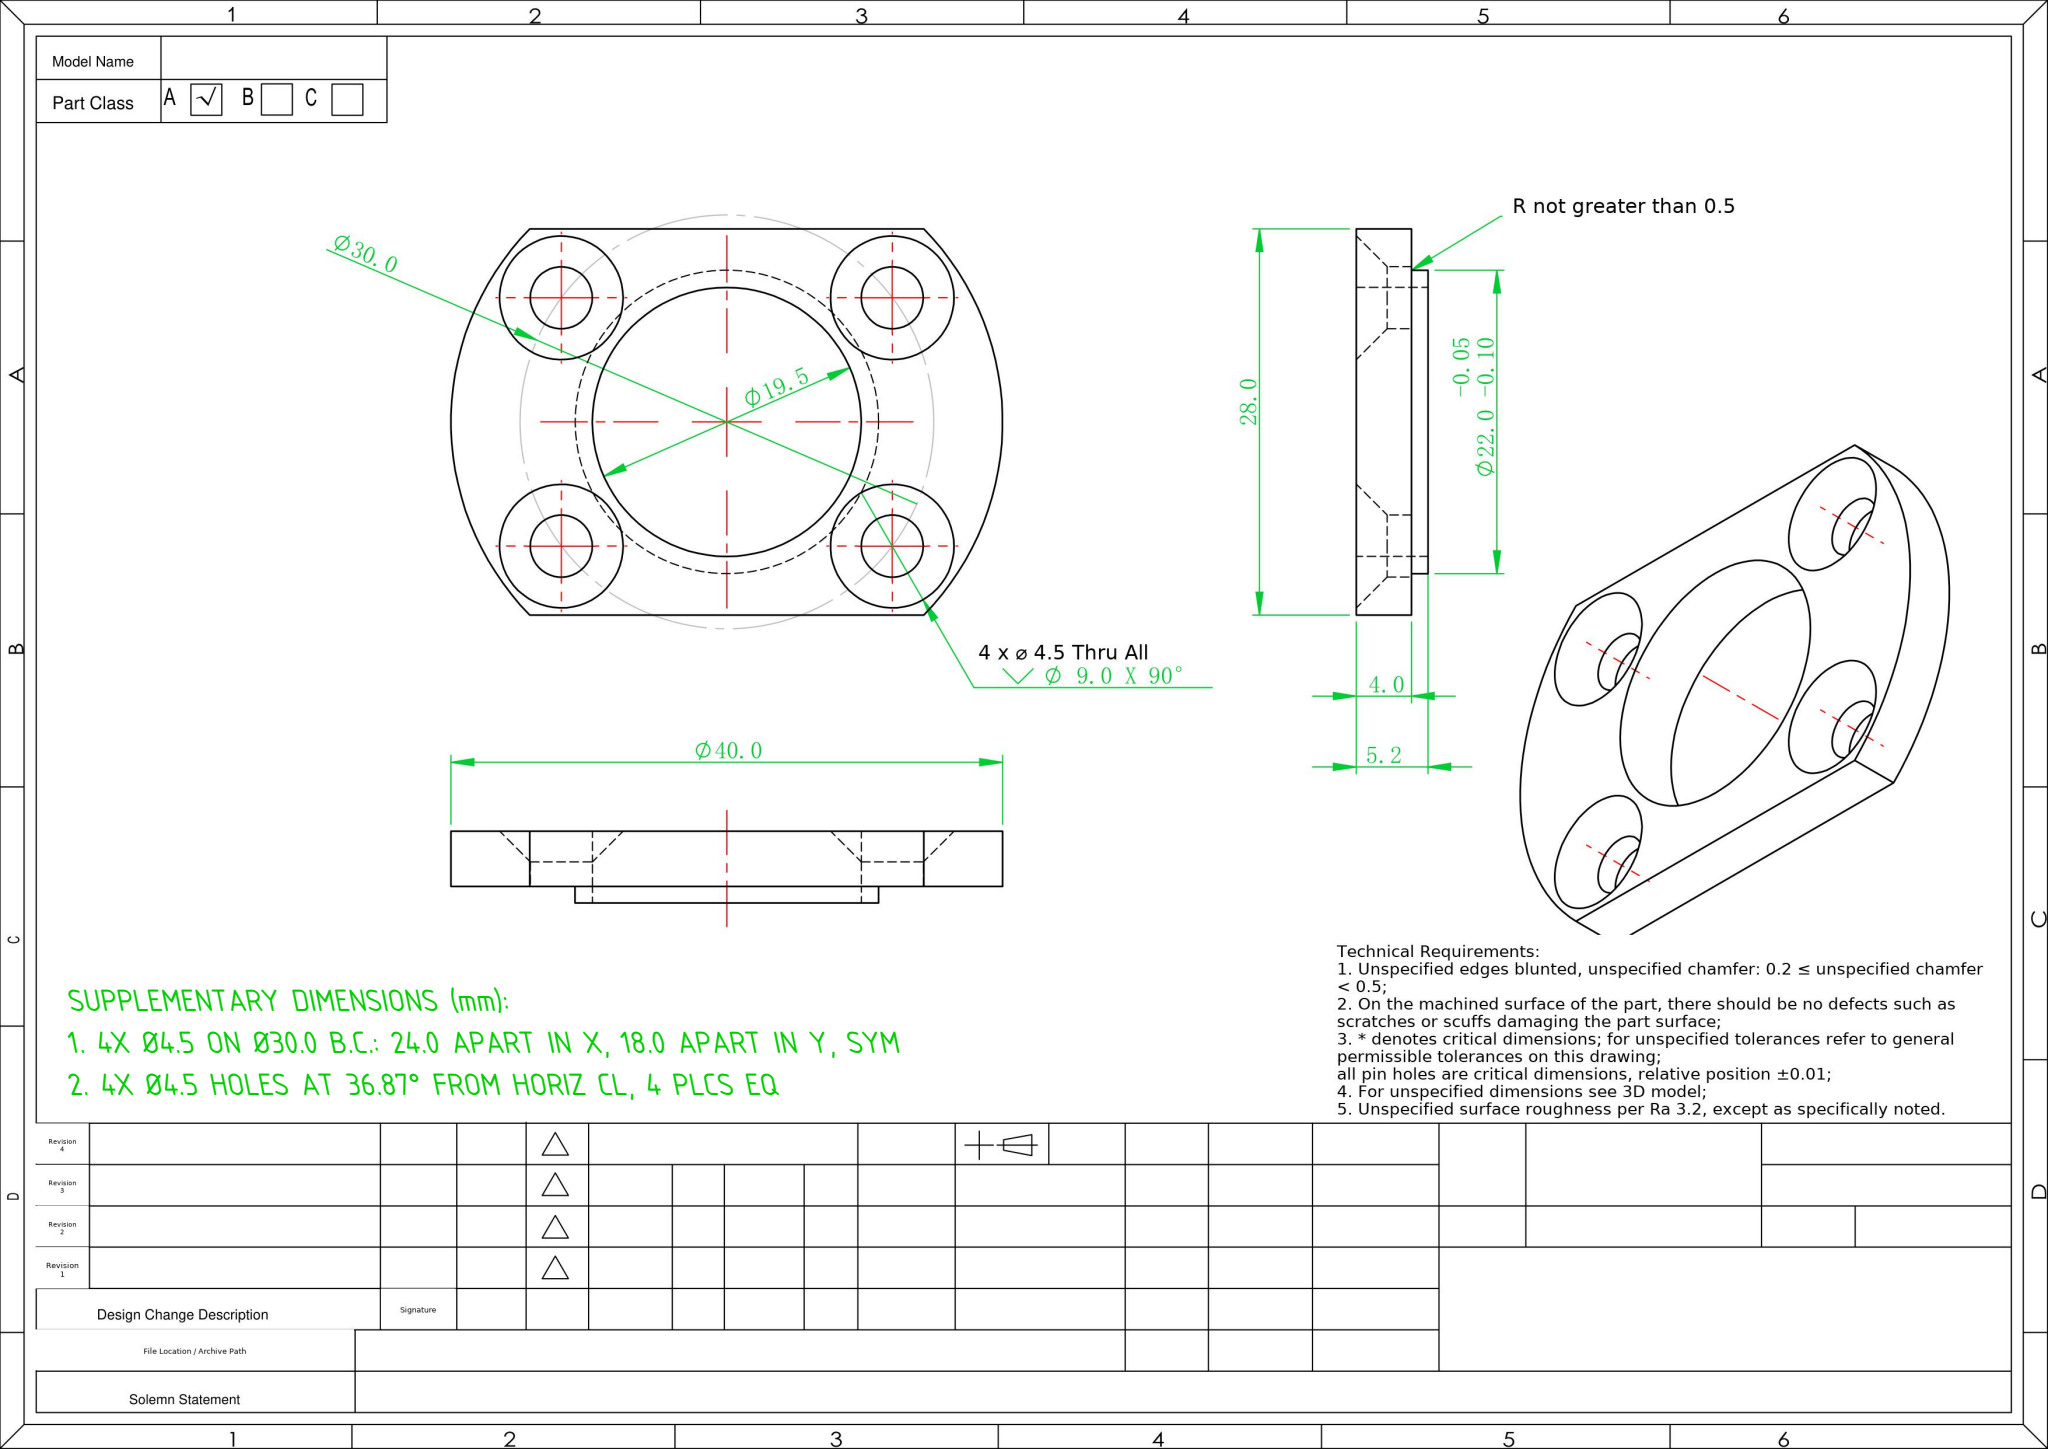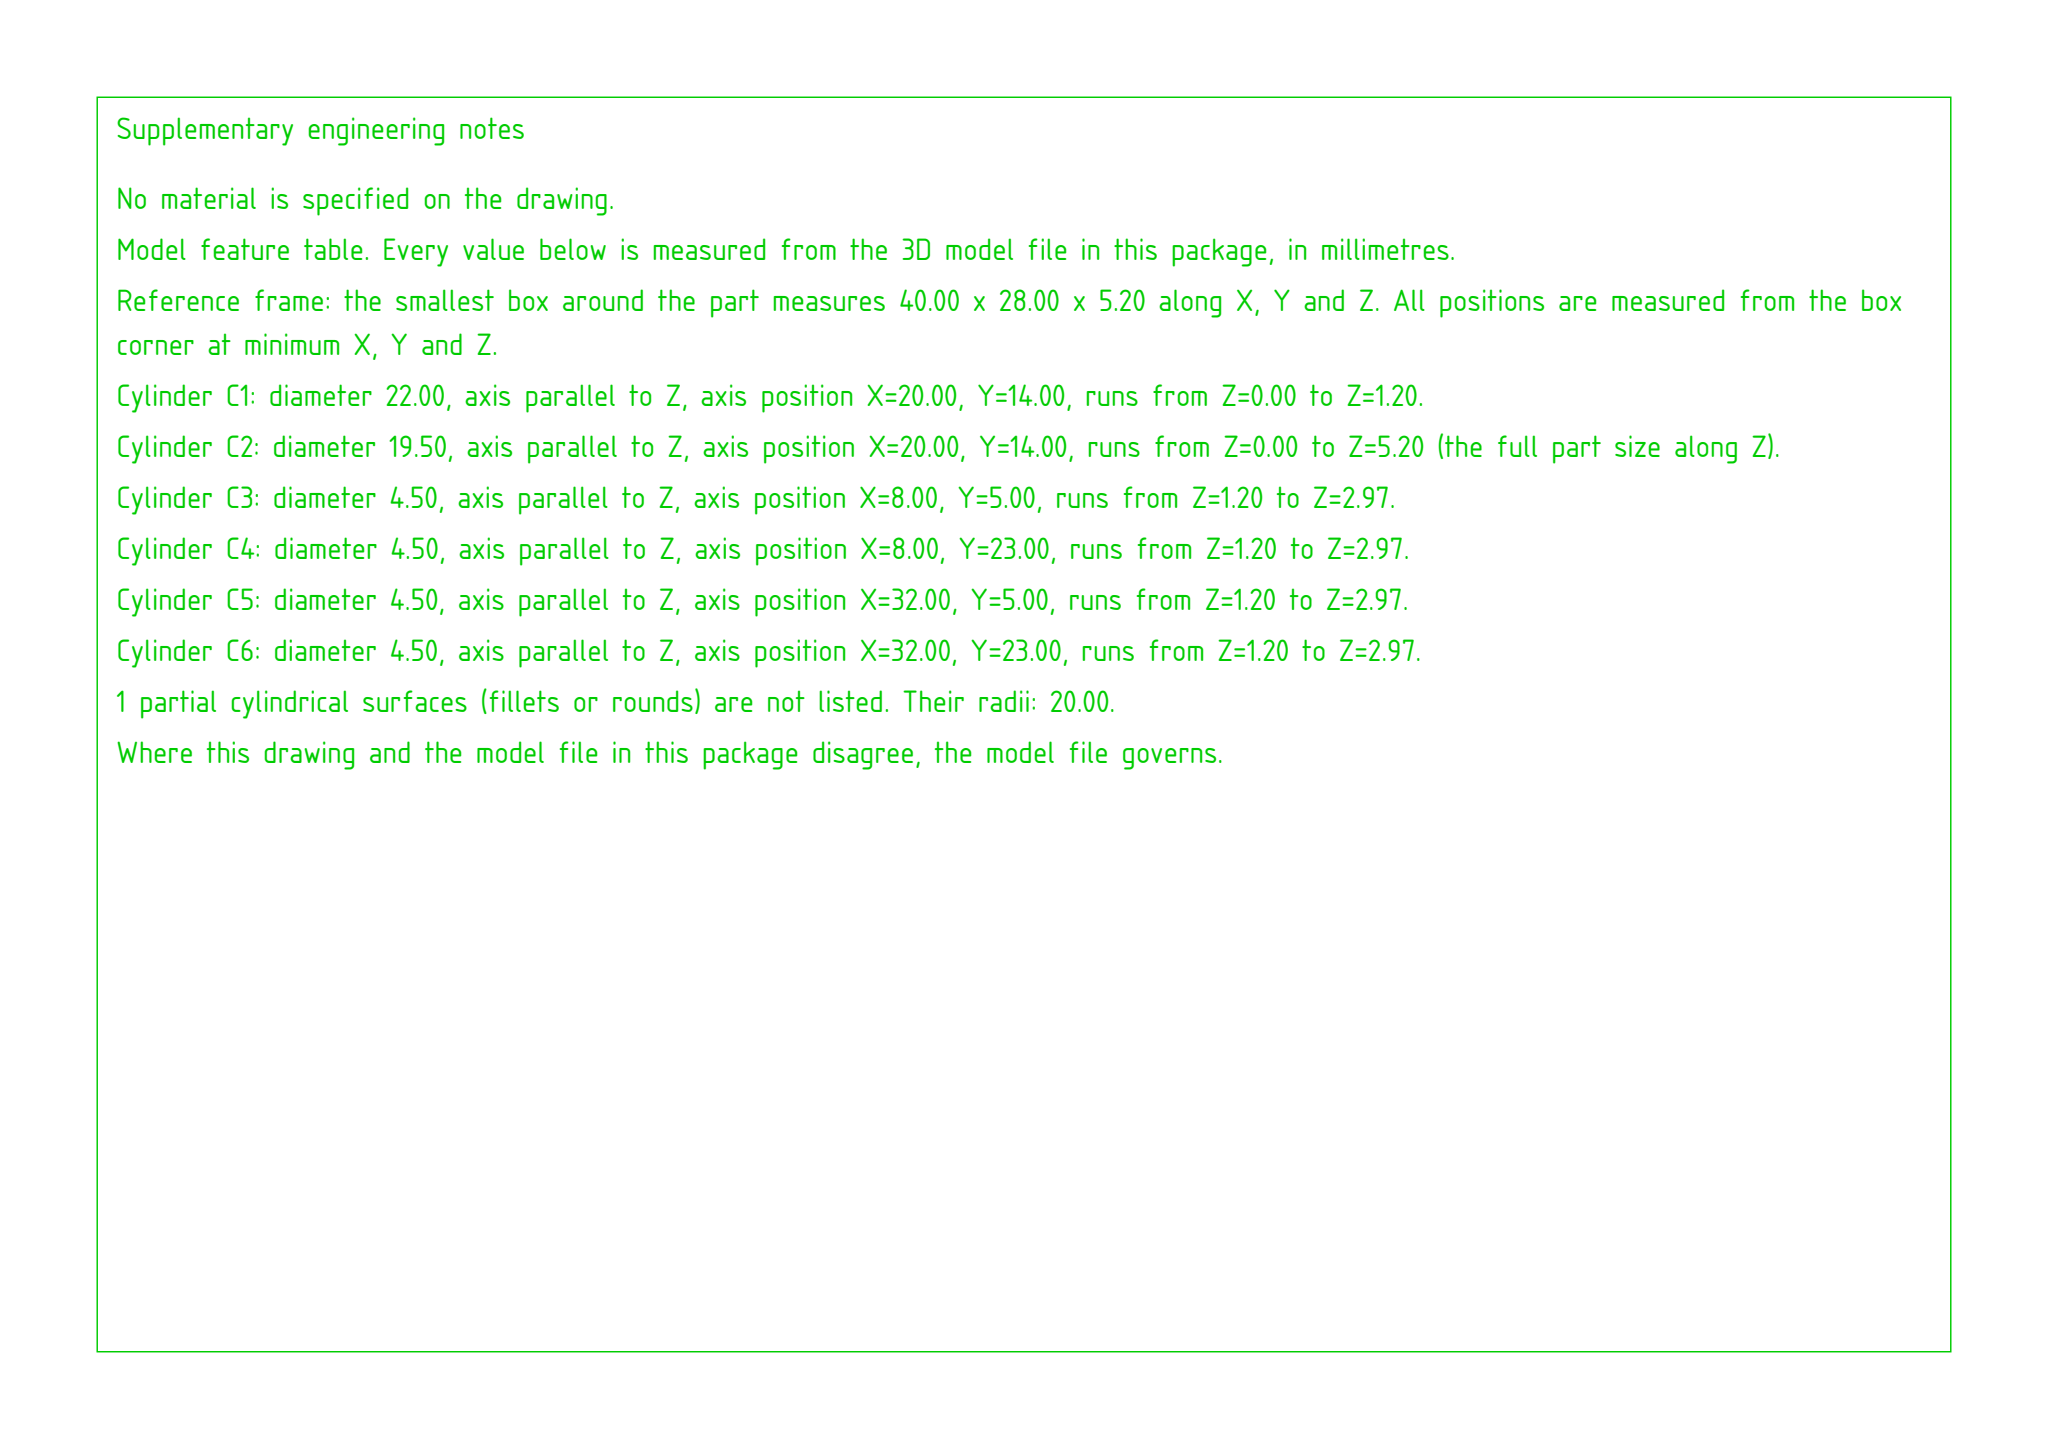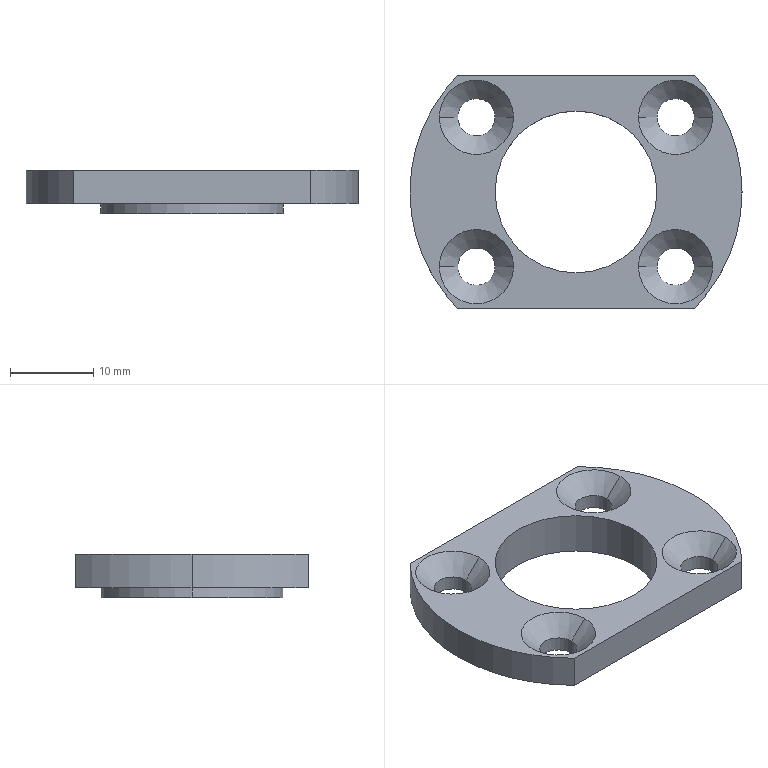Part | SolidWorks | mm | 1 solid | 28 faces | box 40 x 28 x 5.2 mm | volume 2543 mm3 | cylinder 15 | cone 8 | plane 5 | commonest cylinder face diameters 4.5 x8 40 x3 19.5 x2 22 x2
build123d program:
from build123d import *

# Parameters (mm, degrees)
SKETCH1_R                                            = 11
BOSS_EXTRUDE1_DEPTH                                  = 1.2
SKETCH2_R                                            = 20
BOSS_EXTRUDE2_DEPTH                                  = 4
SKETCH3_R                                            = 9.75
CUT_EXTRUDE1_DEPTH                                   = 29.758
SKETCH4_W                                            = 35.499
SKETCH4_H                                            = 10
CUT_EXTRUDE5_DEPTH                                   = 10
COUNTERSUNK_HOLE_FOR_M4_HEXAGON_SOCKET_C_D           = 4.5
COUNTERSUNK_HOLE_FOR_M4_HEXAGON_SOCKET_C_CSINK_D     = 8.96
COUNTERSUNK_HOLE_FOR_M4_HEXAGON_SOCKET_C_CSINK_ANGLE = 90


with BuildPart() as part:
    # Sketch1 → Boss-Extrude1 (new body)
    with BuildSketch(Plane.XY):
        Circle(SKETCH1_R)
    extrude(amount=BOSS_EXTRUDE1_DEPTH)

    # Sketch2 → Boss-Extrude2 (add)
    with BuildSketch(Plane.XY.offset(1.2)):
        Circle(SKETCH2_R)
    extrude(amount=BOSS_EXTRUDE2_DEPTH)

    # Sketch3 → Cut-Extrude1 (cut, through all)
    with BuildSketch(Plane.XY.offset(5.2)):
        Circle(SKETCH3_R)
    extrude(amount=-CUT_EXTRUDE1_DEPTH, mode=Mode.SUBTRACT)

    # Sketch4 → Cut-Extrude5 (cut)
    with BuildSketch(Plane.XY.offset(5.2)):
        with Locations((0, 19)):
            Rectangle(SKETCH4_W, SKETCH4_H)
        with Locations((0, -19)):
            Rectangle(SKETCH4_W, SKETCH4_H)
    extrude(amount=-CUT_EXTRUDE5_DEPTH, mode=Mode.SUBTRACT)

    # Countersunk Hole for M4 Hexagon Socket C (through all)
    with Locations(Plane.XY.offset(5.2)):
        with Locations((-12, 9), (-12, -9), (12, -9), (12, 9)):
            CounterSinkHole(COUNTERSUNK_HOLE_FOR_M4_HEXAGON_SOCKET_C_D / 2, COUNTERSUNK_HOLE_FOR_M4_HEXAGON_SOCKET_C_CSINK_D / 2, counter_sink_angle=COUNTERSUNK_HOLE_FOR_M4_HEXAGON_SOCKET_C_CSINK_ANGLE)


solid = part.part
STEP:
#1=CARTESIAN_POINT('',(-14.25,9.,2.97));
#2=VERTEX_POINT('',#1);
#3=CARTESIAN_POINT('',(-9.75,9.,2.97));
#4=VERTEX_POINT('',#3);
#5=CARTESIAN_POINT('',(-12.,9.,2.97));
#6=DIRECTION('',(0.,0.,1.));
#7=DIRECTION('',(1.,0.,0.));
#8=AXIS2_PLACEMENT_3D('',#5,#6,#7);
#9=CIRCLE('',#8,2.25);
#10=EDGE_CURVE('',#2,#4,#9,.T.);
#11=ORIENTED_EDGE('',*,*,#10,.F.);
#12=CARTESIAN_POINT('',(-16.48,9.,5.2));
#13=VERTEX_POINT('',#12);
#14=CARTESIAN_POINT('',(-16.48,9.,5.2));
#15=DIRECTION('',(-0.7071,0.,0.7071));
#16=VECTOR('',#15,1000.);
#17=LINE('',#14,#16);
#18=EDGE_CURVE('',#2,#13,#17,.T.);
#19=ORIENTED_EDGE('',*,*,#18,.T.);
#20=CARTESIAN_POINT('',(-7.52,9.,5.2));
#21=VERTEX_POINT('',#20);
#22=CARTESIAN_POINT('',(-12.,9.,5.2));
#23=DIRECTION('',(0.,0.,1.));
#24=DIRECTION('',(1.,0.,0.));
#25=AXIS2_PLACEMENT_3D('',#22,#23,#24);
#26=CIRCLE('',#25,4.48);
#27=EDGE_CURVE('',#13,#21,#26,.T.);
#28=ORIENTED_EDGE('',*,*,#27,.T.);
#29=CARTESIAN_POINT('',(-7.52,9.,5.2));
#30=DIRECTION('',(0.7071,0.,0.7071));
#31=VECTOR('',#30,1000.);
#32=LINE('',#29,#31);
#33=EDGE_CURVE('',#4,#21,#32,.T.);
#34=ORIENTED_EDGE('',*,*,#33,.F.);
#35=EDGE_LOOP('',(#11,#19,#28,#34));
#36=FACE_OUTER_BOUND('',#35,.T.);
#37=CARTESIAN_POINT('',(-12.,9.,5.2));
#38=DIRECTION('',(0.,0.,1.));
#39=DIRECTION('',(1.,0.,0.));
#40=AXIS2_PLACEMENT_3D('',#37,#38,#39);
#41=CONICAL_SURFACE('',#40,4.48,0.7854);
#42=ADVANCED_FACE('',(#36),#41,.F.);
#43=CARTESIAN_POINT('',(-14.25,9.,1.2));
#44=VERTEX_POINT('',#43);
#45=CARTESIAN_POINT('',(-9.75,9.,1.2));
#46=VERTEX_POINT('',#45);
#47=CARTESIAN_POINT('',(-12.,9.,1.2));
#48=DIRECTION('',(0.,0.,1.));
#49=DIRECTION('',(1.,0.,0.));
#50=AXIS2_PLACEMENT_3D('',#47,#48,#49);
#51=CIRCLE('',#50,2.25);
#52=EDGE_CURVE('',#44,#46,#51,.T.);
#53=ORIENTED_EDGE('',*,*,#52,.F.);
#54=CARTESIAN_POINT('',(-14.25,9.,5.2));
#55=DIRECTION('',(0.,0.,1.));
#56=VECTOR('',#55,1000.);
#57=LINE('',#54,#56);
#58=EDGE_CURVE('',#44,#2,#57,.T.);
#59=ORIENTED_EDGE('',*,*,#58,.T.);
#60=ORIENTED_EDGE('',*,*,#10,.T.);
#61=CARTESIAN_POINT('',(-9.75,9.,5.2));
#62=DIRECTION('',(0.,0.,1.));
#63=VECTOR('',#62,1000.);
#64=LINE('',#61,#63);
#65=EDGE_CURVE('',#46,#4,#64,.T.);
#66=ORIENTED_EDGE('',*,*,#65,.F.);
#67=EDGE_LOOP('',(#53,#59,#60,#66));
#68=FACE_OUTER_BOUND('',#67,.T.);
#69=CARTESIAN_POINT('',(-12.,9.,5.2));
#70=DIRECTION('',(0.,0.,1.));
#71=DIRECTION('',(1.,0.,0.));
#72=AXIS2_PLACEMENT_3D('',#69,#70,#71);
#73=CYLINDRICAL_SURFACE('',#72,2.25);
#74=ADVANCED_FACE('',(#68),#73,.F.);
#75=CARTESIAN_POINT('',(-14.25,-9.,2.97));
#76=VERTEX_POINT('',#75);
#77=CARTESIAN_POINT('',(-9.75,-9.,2.97));
#78=VERTEX_POINT('',#77);
#79=CARTESIAN_POINT('',(-12.,-9.,2.97));
#80=DIRECTION('',(0.,0.,1.));
#81=DIRECTION('',(1.,0.,0.));
#82=AXIS2_PLACEMENT_3D('',#79,#80,#81);
#83=CIRCLE('',#82,2.25);
#84=EDGE_CURVE('',#76,#78,#83,.T.);
#85=ORIENTED_EDGE('',*,*,#84,.F.);
#86=CARTESIAN_POINT('',(-16.48,-9.,5.2));
#87=VERTEX_POINT('',#86);
#88=CARTESIAN_POINT('',(-16.48,-9.,5.2));
#89=DIRECTION('',(-0.7071,0.,0.7071));
#90=VECTOR('',#89,1000.);
#91=LINE('',#88,#90);
#92=EDGE_CURVE('',#76,#87,#91,.T.);
#93=ORIENTED_EDGE('',*,*,#92,.T.);
#94=CARTESIAN_POINT('',(-7.52,-9.,5.2));
#95=VERTEX_POINT('',#94);
#96=CARTESIAN_POINT('',(-12.,-9.,5.2));
#97=DIRECTION('',(0.,0.,1.));
#98=DIRECTION('',(1.,0.,0.));
#99=AXIS2_PLACEMENT_3D('',#96,#97,#98);
#100=CIRCLE('',#99,4.48);
#101=EDGE_CURVE('',#87,#95,#100,.T.);
#102=ORIENTED_EDGE('',*,*,#101,.T.);
#103=CARTESIAN_POINT('',(-7.52,-9.,5.2));
#104=DIRECTION('',(0.7071,0.,0.7071));
#105=VECTOR('',#104,1000.);
#106=LINE('',#103,#105);
#107=EDGE_CURVE('',#78,#95,#106,.T.);
#108=ORIENTED_EDGE('',*,*,#107,.F.);
#109=EDGE_LOOP('',(#85,#93,#102,#108));
#110=FACE_OUTER_BOUND('',#109,.T.);
#111=CARTESIAN_POINT('',(-12.,-9.,5.2));
#112=DIRECTION('',(0.,0.,1.));
#113=DIRECTION('',(1.,0.,0.));
#114=AXIS2_PLACEMENT_3D('',#111,#112,#113);
#115=CONICAL_SURFACE('',#114,4.48,0.7854);
#116=ADVANCED_FACE('',(#110),#115,.F.);
#117=CARTESIAN_POINT('',(-14.25,-9.,1.2));
#118=VERTEX_POINT('',#117);
#119=CARTESIAN_POINT('',(-9.75,-9.,1.2));
#120=VERTEX_POINT('',#119);
#121=CARTESIAN_POINT('',(-12.,-9.,1.2));
#122=DIRECTION('',(0.,0.,1.));
#123=DIRECTION('',(1.,0.,0.));
#124=AXIS2_PLACEMENT_3D('',#121,#122,#123);
#125=CIRCLE('',#124,2.25);
#126=EDGE_CURVE('',#118,#120,#125,.T.);
#127=ORIENTED_EDGE('',*,*,#126,.F.);
#128=CARTESIAN_POINT('',(-14.25,-9.,5.2));
#129=DIRECTION('',(0.,0.,1.));
#130=VECTOR('',#129,1000.);
#131=LINE('',#128,#130);
#132=EDGE_CURVE('',#118,#76,#131,.T.);
#133=ORIENTED_EDGE('',*,*,#132,.T.);
#134=ORIENTED_EDGE('',*,*,#84,.T.);
#135=CARTESIAN_POINT('',(-9.75,-9.,5.2));
#136=DIRECTION('',(0.,0.,1.));
#137=VECTOR('',#136,1000.);
#138=LINE('',#135,#137);
#139=EDGE_CURVE('',#120,#78,#138,.T.);
#140=ORIENTED_EDGE('',*,*,#139,.F.);
#141=EDGE_LOOP('',(#127,#133,#134,#140));
#142=FACE_OUTER_BOUND('',#141,.T.);
#143=CARTESIAN_POINT('',(-12.,-9.,5.2));
#144=DIRECTION('',(0.,0.,1.));
#145=DIRECTION('',(1.,0.,0.));
#146=AXIS2_PLACEMENT_3D('',#143,#144,#145);
#147=CYLINDRICAL_SURFACE('',#146,2.25);
#148=ADVANCED_FACE('',(#142),#147,.F.);
#149=CARTESIAN_POINT('',(9.75,-9.,2.97));
#150=VERTEX_POINT('',#149);
#151=CARTESIAN_POINT('',(14.25,-9.,2.97));
#152=VERTEX_POINT('',#151);
#153=CARTESIAN_POINT('',(12.,-9.,2.97));
#154=DIRECTION('',(0.,0.,1.));
#155=DIRECTION('',(1.,0.,0.));
#156=AXIS2_PLACEMENT_3D('',#153,#154,#155);
#157=CIRCLE('',#156,2.25);
#158=EDGE_CURVE('',#150,#152,#157,.T.);
#159=ORIENTED_EDGE('',*,*,#158,.F.);
#160=CARTESIAN_POINT('',(7.52,-9.,5.2));
#161=VERTEX_POINT('',#160);
#162=CARTESIAN_POINT('',(7.52,-9.,5.2));
#163=DIRECTION('',(-0.7071,0.,0.7071));
#164=VECTOR('',#163,1000.);
#165=LINE('',#162,#164);
#166=EDGE_CURVE('',#150,#161,#165,.T.);
#167=ORIENTED_EDGE('',*,*,#166,.T.);
#168=CARTESIAN_POINT('',(16.48,-9.,5.2));
#169=VERTEX_POINT('',#168);
#170=CARTESIAN_POINT('',(12.,-9.,5.2));
#171=DIRECTION('',(0.,0.,1.));
#172=DIRECTION('',(1.,0.,0.));
#173=AXIS2_PLACEMENT_3D('',#170,#171,#172);
#174=CIRCLE('',#173,4.48);
#175=EDGE_CURVE('',#161,#169,#174,.T.);
#176=ORIENTED_EDGE('',*,*,#175,.T.);
#177=CARTESIAN_POINT('',(16.48,-9.,5.2));
#178=DIRECTION('',(0.7071,0.,0.7071));
#179=VECTOR('',#178,1000.);
#180=LINE('',#177,#179);
#181=EDGE_CURVE('',#152,#169,#180,.T.);
#182=ORIENTED_EDGE('',*,*,#181,.F.);
#183=EDGE_LOOP('',(#159,#167,#176,#182));
#184=FACE_OUTER_BOUND('',#183,.T.);
#185=CARTESIAN_POINT('',(12.,-9.,5.2));
#186=DIRECTION('',(0.,0.,1.));
#187=DIRECTION('',(1.,0.,0.));
#188=AXIS2_PLACEMENT_3D('',#185,#186,#187);
#189=CONICAL_SURFACE('',#188,4.48,0.7854);
#190=ADVANCED_FACE('',(#184),#189,.F.);
#191=CARTESIAN_POINT('',(9.75,-9.,1.2));
#192=VERTEX_POINT('',#191);
#193=CARTESIAN_POINT('',(14.25,-9.,1.2));
#194=VERTEX_POINT('',#193);
#195=CARTESIAN_POINT('',(12.,-9.,1.2));
#196=DIRECTION('',(0.,0.,1.));
#197=DIRECTION('',(1.,0.,0.));
#198=AXIS2_PLACEMENT_3D('',#195,#196,#197);
#199=CIRCLE('',#198,2.25);
#200=EDGE_CURVE('',#192,#194,#199,.T.);
#201=ORIENTED_EDGE('',*,*,#200,.F.);
#202=CARTESIAN_POINT('',(9.75,-9.,5.2));
#203=DIRECTION('',(0.,0.,1.));
#204=VECTOR('',#203,1000.);
#205=LINE('',#202,#204);
#206=EDGE_CURVE('',#192,#150,#205,.T.);
#207=ORIENTED_EDGE('',*,*,#206,.T.);
#208=ORIENTED_EDGE('',*,*,#158,.T.);
#209=CARTESIAN_POINT('',(14.25,-9.,5.2));
#210=DIRECTION('',(0.,0.,1.));
#211=VECTOR('',#210,1000.);
#212=LINE('',#209,#211);
#213=EDGE_CURVE('',#194,#152,#212,.T.);
#214=ORIENTED_EDGE('',*,*,#213,.F.);
#215=EDGE_LOOP('',(#201,#207,#208,#214));
#216=FACE_OUTER_BOUND('',#215,.T.);
#217=CARTESIAN_POINT('',(12.,-9.,5.2));
#218=DIRECTION('',(0.,0.,1.));
#219=DIRECTION('',(1.,0.,0.));
#220=AXIS2_PLACEMENT_3D('',#217,#218,#219);
#221=CYLINDRICAL_SURFACE('',#220,2.25);
#222=ADVANCED_FACE('',(#216),#221,.F.);
#223=CARTESIAN_POINT('',(9.75,9.,2.97));
#224=VERTEX_POINT('',#223);
#225=CARTESIAN_POINT('',(14.25,9.,2.97));
#226=VERTEX_POINT('',#225);
#227=CARTESIAN_POINT('',(12.,9.,2.97));
#228=DIRECTION('',(0.,0.,1.));
#229=DIRECTION('',(1.,0.,0.));
#230=AXIS2_PLACEMENT_3D('',#227,#228,#229);
#231=CIRCLE('',#230,2.25);
#232=EDGE_CURVE('',#224,#226,#231,.T.);
#233=ORIENTED_EDGE('',*,*,#232,.F.);
#234=CARTESIAN_POINT('',(7.52,9.,5.2));
#235=VERTEX_POINT('',#234);
#236=CARTESIAN_POINT('',(7.52,9.,5.2));
#237=DIRECTION('',(-0.7071,0.,0.7071));
#238=VECTOR('',#237,1000.);
#239=LINE('',#236,#238);
#240=EDGE_CURVE('',#224,#235,#239,.T.);
#241=ORIENTED_EDGE('',*,*,#240,.T.);
#242=CARTESIAN_POINT('',(16.48,9.,5.2));
#243=VERTEX_POINT('',#242);
#244=CARTESIAN_POINT('',(12.,9.,5.2));
#245=DIRECTION('',(0.,0.,1.));
#246=DIRECTION('',(1.,0.,0.));
#247=AXIS2_PLACEMENT_3D('',#244,#245,#246);
#248=CIRCLE('',#247,4.48);
#249=EDGE_CURVE('',#235,#243,#248,.T.);
#250=ORIENTED_EDGE('',*,*,#249,.T.);
#251=CARTESIAN_POINT('',(16.48,9.,5.2));
#252=DIRECTION('',(0.7071,0.,0.7071));
#253=VECTOR('',#252,1000.);
#254=LINE('',#251,#253);
#255=EDGE_CURVE('',#226,#243,#254,.T.);
#256=ORIENTED_EDGE('',*,*,#255,.F.);
#257=EDGE_LOOP('',(#233,#241,#250,#256));
#258=FACE_OUTER_BOUND('',#257,.T.);
#259=CARTESIAN_POINT('',(12.,9.,5.2));
#260=DIRECTION('',(0.,0.,1.));
#261=DIRECTION('',(1.,0.,0.));
#262=AXIS2_PLACEMENT_3D('',#259,#260,#261);
#263=CONICAL_SURFACE('',#262,4.48,0.7854);
#264=ADVANCED_FACE('',(#258),#263,.F.);
#265=CARTESIAN_POINT('',(9.75,9.,1.2));
#266=VERTEX_POINT('',#265);
#267=CARTESIAN_POINT('',(14.25,9.,1.2));
#268=VERTEX_POINT('',#267);
#269=CARTESIAN_POINT('',(12.,9.,1.2));
#270=DIRECTION('',(0.,0.,1.));
#271=DIRECTION('',(1.,0.,0.));
#272=AXIS2_PLACEMENT_3D('',#269,#270,#271);
#273=CIRCLE('',#272,2.25);
#274=EDGE_CURVE('',#266,#268,#273,.T.);
#275=ORIENTED_EDGE('',*,*,#274,.F.);
#276=CARTESIAN_POINT('',(9.75,9.,5.2));
#277=DIRECTION('',(0.,0.,1.));
#278=VECTOR('',#277,1000.);
#279=LINE('',#276,#278);
#280=EDGE_CURVE('',#266,#224,#279,.T.);
#281=ORIENTED_EDGE('',*,*,#280,.T.);
#282=ORIENTED_EDGE('',*,*,#232,.T.);
#283=CARTESIAN_POINT('',(14.25,9.,5.2));
#284=DIRECTION('',(0.,0.,1.));
#285=VECTOR('',#284,1000.);
#286=LINE('',#283,#285);
#287=EDGE_CURVE('',#268,#226,#286,.T.);
#288=ORIENTED_EDGE('',*,*,#287,.F.);
#289=EDGE_LOOP('',(#275,#281,#282,#288));
#290=FACE_OUTER_BOUND('',#289,.T.);
#291=CARTESIAN_POINT('',(12.,9.,5.2));
#292=DIRECTION('',(0.,0.,1.));
#293=DIRECTION('',(1.,0.,0.));
#294=AXIS2_PLACEMENT_3D('',#291,#292,#293);
#295=CYLINDRICAL_SURFACE('',#294,2.25);
#296=ADVANCED_FACE('',(#290),#295,.F.);
#297=CARTESIAN_POINT('',(-9.75,0.,0.));
#298=VERTEX_POINT('',#297);
#299=CARTESIAN_POINT('',(9.75,0.,0.));
#300=VERTEX_POINT('',#299);
#301=CARTESIAN_POINT('',(0.,0.,0.));
#302=DIRECTION('',(0.,0.,1.));
#303=DIRECTION('',(1.,0.,0.));
#304=AXIS2_PLACEMENT_3D('',#301,#302,#303);
#305=CIRCLE('',#304,9.75);
#306=EDGE_CURVE('',#298,#300,#305,.T.);
#307=ORIENTED_EDGE('',*,*,#306,.F.);
#308=CARTESIAN_POINT('',(-9.75,0.,5.2));
#309=VERTEX_POINT('',#308);
#310=CARTESIAN_POINT('',(-9.75,0.,0.));
#311=DIRECTION('',(0.,0.,1.));
#312=VECTOR('',#311,1000.);
#313=LINE('',#310,#312);
#314=EDGE_CURVE('',#298,#309,#313,.T.);
#315=ORIENTED_EDGE('',*,*,#314,.T.);
#316=CARTESIAN_POINT('',(9.75,0.,5.2));
#317=VERTEX_POINT('',#316);
#318=CARTESIAN_POINT('',(0.,0.,5.2));
#319=DIRECTION('',(0.,0.,1.));
#320=DIRECTION('',(1.,0.,0.));
#321=AXIS2_PLACEMENT_3D('',#318,#319,#320);
#322=CIRCLE('',#321,9.75);
#323=EDGE_CURVE('',#309,#317,#322,.T.);
#324=ORIENTED_EDGE('',*,*,#323,.T.);
#325=CARTESIAN_POINT('',(9.75,0.,0.));
#326=DIRECTION('',(0.,0.,1.));
#327=VECTOR('',#326,1000.);
#328=LINE('',#325,#327);
#329=EDGE_CURVE('',#300,#317,#328,.T.);
#330=ORIENTED_EDGE('',*,*,#329,.F.);
#331=EDGE_LOOP('',(#307,#315,#324,#330));
#332=FACE_OUTER_BOUND('',#331,.T.);
#333=CARTESIAN_POINT('',(0.,0.,0.));
#334=DIRECTION('',(0.,0.,1.));
#335=DIRECTION('',(1.,0.,0.));
#336=AXIS2_PLACEMENT_3D('',#333,#334,#335);
#337=CYLINDRICAL_SURFACE('',#336,9.75);
#338=ADVANCED_FACE('',(#332),#337,.F.);
#339=CARTESIAN_POINT('',(11.,0.,1.2));
#340=VERTEX_POINT('',#339);
#341=CARTESIAN_POINT('',(-11.,0.,1.2));
#342=VERTEX_POINT('',#341);
#343=CARTESIAN_POINT('',(0.,0.,1.2));
#344=DIRECTION('',(0.,0.,1.));
#345=DIRECTION('',(1.,0.,0.));
#346=AXIS2_PLACEMENT_3D('',#343,#344,#345);
#347=CIRCLE('',#346,11.);
#348=EDGE_CURVE('',#340,#342,#347,.T.);
#349=ORIENTED_EDGE('',*,*,#348,.F.);
#350=CARTESIAN_POINT('',(11.,0.,0.));
#351=VERTEX_POINT('',#350);
#352=CARTESIAN_POINT('',(11.,0.,1.2));
#353=DIRECTION('',(0.,0.,-1.));
#354=VECTOR('',#353,1000.);
#355=LINE('',#352,#354);
#356=EDGE_CURVE('',#340,#351,#355,.T.);
#357=ORIENTED_EDGE('',*,*,#356,.T.);
#358=CARTESIAN_POINT('',(-11.,0.,0.));
#359=VERTEX_POINT('',#358);
#360=CARTESIAN_POINT('',(0.,0.,0.));
#361=DIRECTION('',(0.,0.,1.));
#362=DIRECTION('',(1.,0.,0.));
#363=AXIS2_PLACEMENT_3D('',#360,#361,#362);
#364=CIRCLE('',#363,11.);
#365=EDGE_CURVE('',#351,#359,#364,.T.);
#366=ORIENTED_EDGE('',*,*,#365,.T.);
#367=CARTESIAN_POINT('',(-11.,0.,1.2));
#368=DIRECTION('',(0.,0.,-1.));
#369=VECTOR('',#368,1000.);
#370=LINE('',#367,#369);
#371=EDGE_CURVE('',#342,#359,#370,.T.);
#372=ORIENTED_EDGE('',*,*,#371,.F.);
#373=EDGE_LOOP('',(#349,#357,#366,#372));
#374=FACE_OUTER_BOUND('',#373,.T.);
#375=CARTESIAN_POINT('',(0.,0.,1.2));
#376=DIRECTION('',(0.,0.,-1.));
#377=DIRECTION('',(-1.,0.,0.));
#378=AXIS2_PLACEMENT_3D('',#375,#376,#377);
#379=CYLINDRICAL_SURFACE('',#378,11.);
#380=ADVANCED_FACE('',(#374),#379,.T.);
#381=CARTESIAN_POINT('',(-20.,0.,5.2));
#382=VERTEX_POINT('',#381);
#383=CARTESIAN_POINT('',(-14.283,-14.,5.2));
#384=VERTEX_POINT('',#383);
#385=CARTESIAN_POINT('',(0.,0.,5.2));
#386=DIRECTION('',(0.,0.,1.));
#387=DIRECTION('',(1.,0.,0.));
#388=AXIS2_PLACEMENT_3D('',#385,#386,#387);
#389=CIRCLE('',#388,20.);
#390=EDGE_CURVE('',#382,#384,#389,.T.);
#391=ORIENTED_EDGE('',*,*,#390,.F.);
#392=CARTESIAN_POINT('',(-20.,0.,1.2));
#393=VERTEX_POINT('',#392);
#394=CARTESIAN_POINT('',(-20.,0.,5.2));
#395=DIRECTION('',(0.,0.,-1.));
#396=VECTOR('',#395,1000.);
#397=LINE('',#394,#396);
#398=EDGE_CURVE('',#382,#393,#397,.T.);
#399=ORIENTED_EDGE('',*,*,#398,.T.);
#400=CARTESIAN_POINT('',(-14.283,-14.,1.2));
#401=VERTEX_POINT('',#400);
#402=CARTESIAN_POINT('',(0.,0.,1.2));
#403=DIRECTION('',(0.,0.,1.));
#404=DIRECTION('',(1.,0.,0.));
#405=AXIS2_PLACEMENT_3D('',#402,#403,#404);
#406=CIRCLE('',#405,20.);
#407=EDGE_CURVE('',#393,#401,#406,.T.);
#408=ORIENTED_EDGE('',*,*,#407,.T.);
#409=CARTESIAN_POINT('',(-14.283,-14.,5.2));
#410=DIRECTION('',(0.,0.,1.));
#411=VECTOR('',#410,1000.);
#412=LINE('',#409,#411);
#413=EDGE_CURVE('',#401,#384,#412,.T.);
#414=ORIENTED_EDGE('',*,*,#413,.T.);
#415=EDGE_LOOP('',(#391,#399,#408,#414));
#416=FACE_OUTER_BOUND('',#415,.T.);
#417=CARTESIAN_POINT('',(0.,0.,5.2));
#418=DIRECTION('',(0.,0.,-1.));
#419=DIRECTION('',(-1.,0.,0.));
#420=AXIS2_PLACEMENT_3D('',#417,#418,#419);
#421=CYLINDRICAL_SURFACE('',#420,20.);
#422=ADVANCED_FACE('',(#416),#421,.T.);
#423=ORIENTED_EDGE('',*,*,#398,.F.);
#424=CARTESIAN_POINT('',(-14.283,14.,5.2));
#425=VERTEX_POINT('',#424);
#426=CARTESIAN_POINT('',(0.,0.,5.2));
#427=DIRECTION('',(0.,0.,1.));
#428=DIRECTION('',(1.,0.,0.));
#429=AXIS2_PLACEMENT_3D('',#426,#427,#428);
#430=CIRCLE('',#429,20.);
#431=EDGE_CURVE('',#425,#382,#430,.T.);
#432=ORIENTED_EDGE('',*,*,#431,.F.);
#433=CARTESIAN_POINT('',(-14.283,14.,1.2));
#434=VERTEX_POINT('',#433);
#435=CARTESIAN_POINT('',(-14.283,14.,5.2));
#436=DIRECTION('',(0.,0.,-1.));
#437=VECTOR('',#436,1000.);
#438=LINE('',#435,#437);
#439=EDGE_CURVE('',#425,#434,#438,.T.);
#440=ORIENTED_EDGE('',*,*,#439,.T.);
#441=CARTESIAN_POINT('',(0.,0.,1.2));
#442=DIRECTION('',(0.,0.,1.));
#443=DIRECTION('',(1.,0.,0.));
#444=AXIS2_PLACEMENT_3D('',#441,#442,#443);
#445=CIRCLE('',#444,20.);
#446=EDGE_CURVE('',#434,#393,#445,.T.);
#447=ORIENTED_EDGE('',*,*,#446,.T.);
#448=EDGE_LOOP('',(#423,#432,#440,#447));
#449=FACE_OUTER_BOUND('',#448,.T.);
#450=CARTESIAN_POINT('',(0.,0.,5.2));
#451=DIRECTION('',(0.,0.,-1.));
#452=DIRECTION('',(-1.,0.,0.));
#453=AXIS2_PLACEMENT_3D('',#450,#451,#452);
#454=CYLINDRICAL_SURFACE('',#453,20.);
#455=ADVANCED_FACE('',(#449),#454,.T.);
#456=ORIENTED_EDGE('',*,*,#356,.F.);
#457=CARTESIAN_POINT('',(0.,0.,1.2));
#458=DIRECTION('',(0.,0.,1.));
#459=DIRECTION('',(1.,0.,0.));
#460=AXIS2_PLACEMENT_3D('',#457,#458,#459);
#461=CIRCLE('',#460,11.);
#462=EDGE_CURVE('',#342,#340,#461,.T.);
#463=ORIENTED_EDGE('',*,*,#462,.F.);
#464=ORIENTED_EDGE('',*,*,#371,.T.);
#465=CARTESIAN_POINT('',(0.,0.,0.));
#466=DIRECTION('',(0.,0.,1.));
#467=DIRECTION('',(1.,0.,0.));
#468=AXIS2_PLACEMENT_3D('',#465,#466,#467);
#469=CIRCLE('',#468,11.);
#470=EDGE_CURVE('',#359,#351,#469,.T.);
#471=ORIENTED_EDGE('',*,*,#470,.T.);
#472=EDGE_LOOP('',(#456,#463,#464,#471));
#473=FACE_OUTER_BOUND('',#472,.T.);
#474=CARTESIAN_POINT('',(0.,0.,1.2));
#475=DIRECTION('',(0.,0.,-1.));
#476=DIRECTION('',(-1.,0.,0.));
#477=AXIS2_PLACEMENT_3D('',#474,#475,#476);
#478=CYLINDRICAL_SURFACE('',#477,11.);
#479=ADVANCED_FACE('',(#473),#478,.T.);
#480=CARTESIAN_POINT('',(0.,0.,0.));
#481=DIRECTION('',(0.,0.,1.));
#482=DIRECTION('',(1.,0.,0.));
#483=AXIS2_PLACEMENT_3D('',#480,#481,#482);
#484=CIRCLE('',#483,9.75);
#485=EDGE_CURVE('',#300,#298,#484,.T.);
#486=ORIENTED_EDGE('',*,*,#485,.T.);
#487=ORIENTED_EDGE('',*,*,#306,.T.);
#488=EDGE_LOOP('',(#486,#487));
#489=FACE_BOUND('',#488,.T.);
#490=ORIENTED_EDGE('',*,*,#470,.F.);
#491=ORIENTED_EDGE('',*,*,#365,.F.);
#492=EDGE_LOOP('',(#490,#491));
#493=FACE_OUTER_BOUND('',#492,.T.);
#494=CARTESIAN_POINT('',(0.,0.,0.));
#495=DIRECTION('',(0.,0.,1.));
#496=DIRECTION('',(1.,0.,0.));
#497=AXIS2_PLACEMENT_3D('',#494,#495,#496);
#498=PLANE('',#497);
#499=ADVANCED_FACE('',(#489,#493),#498,.F.);
#500=CARTESIAN_POINT('',(14.283,-14.,1.2));
#501=VERTEX_POINT('',#500);
#502=CARTESIAN_POINT('',(14.283,14.,1.2));
#503=VERTEX_POINT('',#502);
#504=CARTESIAN_POINT('',(0.,0.,1.2));
#505=DIRECTION('',(0.,0.,1.));
#506=DIRECTION('',(1.,0.,0.));
#507=AXIS2_PLACEMENT_3D('',#504,#505,#506);
#508=CIRCLE('',#507,20.);
#509=EDGE_CURVE('',#501,#503,#508,.T.);
#510=ORIENTED_EDGE('',*,*,#509,.T.);
#511=CARTESIAN_POINT('',(14.283,14.,5.2));
#512=VERTEX_POINT('',#511);
#513=CARTESIAN_POINT('',(14.283,14.,5.2));
#514=DIRECTION('',(0.,0.,1.));
#515=VECTOR('',#514,1000.);
#516=LINE('',#513,#515);
#517=EDGE_CURVE('',#503,#512,#516,.T.);
#518=ORIENTED_EDGE('',*,*,#517,.T.);
#519=CARTESIAN_POINT('',(14.283,-14.,5.2));
#520=VERTEX_POINT('',#519);
#521=CARTESIAN_POINT('',(0.,0.,5.2));
#522=DIRECTION('',(0.,0.,1.));
#523=DIRECTION('',(1.,0.,0.));
#524=AXIS2_PLACEMENT_3D('',#521,#522,#523);
#525=CIRCLE('',#524,20.);
#526=EDGE_CURVE('',#520,#512,#525,.T.);
#527=ORIENTED_EDGE('',*,*,#526,.F.);
#528=CARTESIAN_POINT('',(14.283,-14.,5.2));
#529=DIRECTION('',(0.,0.,-1.));
#530=VECTOR('',#529,1000.);
#531=LINE('',#528,#530);
#532=EDGE_CURVE('',#520,#501,#531,.T.);
#533=ORIENTED_EDGE('',*,*,#532,.T.);
#534=EDGE_LOOP('',(#510,#518,#527,#533));
#535=FACE_OUTER_BOUND('',#534,.T.);
#536=CARTESIAN_POINT('',(0.,0.,5.2));
#537=DIRECTION('',(0.,0.,-1.));
#538=DIRECTION('',(-1.,0.,0.));
#539=AXIS2_PLACEMENT_3D('',#536,#537,#538);
#540=CYLINDRICAL_SURFACE('',#539,20.);
#541=ADVANCED_FACE('',(#535),#540,.T.);
#542=CARTESIAN_POINT('',(-12.,9.,5.2));
#543=DIRECTION('',(0.,0.,1.));
#544=DIRECTION('',(1.,0.,0.));
#545=AXIS2_PLACEMENT_3D('',#542,#543,#544);
#546=CIRCLE('',#545,4.48);
#547=EDGE_CURVE('',#21,#13,#546,.T.);
#548=ORIENTED_EDGE('',*,*,#547,.F.);
#549=ORIENTED_EDGE('',*,*,#27,.F.);
#550=EDGE_LOOP('',(#548,#549));
#551=FACE_BOUND('',#550,.T.);
#552=CARTESIAN_POINT('',(-12.,-9.,5.2));
#553=DIRECTION('',(0.,0.,1.));
#554=DIRECTION('',(1.,0.,0.));
#555=AXIS2_PLACEMENT_3D('',#552,#553,#554);
#556=CIRCLE('',#555,4.48);
#557=EDGE_CURVE('',#95,#87,#556,.T.);
#558=ORIENTED_EDGE('',*,*,#557,.F.);
#559=ORIENTED_EDGE('',*,*,#101,.F.);
#560=EDGE_LOOP('',(#558,#559));
#561=FACE_BOUND('',#560,.T.);
#562=CARTESIAN_POINT('',(12.,-9.,5.2));
#563=DIRECTION('',(0.,0.,1.));
#564=DIRECTION('',(1.,0.,0.));
#565=AXIS2_PLACEMENT_3D('',#562,#563,#564);
#566=CIRCLE('',#565,4.48);
#567=EDGE_CURVE('',#169,#161,#566,.T.);
#568=ORIENTED_EDGE('',*,*,#567,.F.);
#569=ORIENTED_EDGE('',*,*,#175,.F.);
#570=EDGE_LOOP('',(#568,#569));
#571=FACE_BOUND('',#570,.T.);
#572=CARTESIAN_POINT('',(12.,9.,5.2));
#573=DIRECTION('',(0.,0.,1.));
#574=DIRECTION('',(1.,0.,0.));
#575=AXIS2_PLACEMENT_3D('',#572,#573,#574);
#576=CIRCLE('',#575,4.48);
#577=EDGE_CURVE('',#243,#235,#576,.T.);
#578=ORIENTED_EDGE('',*,*,#577,.F.);
#579=ORIENTED_EDGE('',*,*,#249,.F.);
#580=EDGE_LOOP('',(#578,#579));
#581=FACE_BOUND('',#580,.T.);
#582=CARTESIAN_POINT('',(-17.749,14.,5.2));
#583=DIRECTION('',(1.,0.,0.));
#584=VECTOR('',#583,1000.);
#585=LINE('',#582,#584);
#586=EDGE_CURVE('',#425,#512,#585,.T.);
#587=ORIENTED_EDGE('',*,*,#586,.F.);
#588=ORIENTED_EDGE('',*,*,#431,.T.);
#589=ORIENTED_EDGE('',*,*,#390,.T.);
#590=CARTESIAN_POINT('',(-17.749,-14.,5.2));
#591=DIRECTION('',(-1.,0.,0.));
#592=VECTOR('',#591,1000.);
#593=LINE('',#590,#592);
#594=EDGE_CURVE('',#520,#384,#593,.T.);
#595=ORIENTED_EDGE('',*,*,#594,.F.);
#596=ORIENTED_EDGE('',*,*,#526,.T.);
#597=EDGE_LOOP('',(#587,#588,#589,#595,#596));
#598=FACE_OUTER_BOUND('',#597,.T.);
#599=CARTESIAN_POINT('',(0.,0.,5.2));
#600=DIRECTION('',(0.,0.,1.));
#601=DIRECTION('',(1.,0.,0.));
#602=AXIS2_PLACEMENT_3D('',#599,#600,#601);
#603=CIRCLE('',#602,9.75);
#604=EDGE_CURVE('',#317,#309,#603,.T.);
#605=ORIENTED_EDGE('',*,*,#604,.F.);
#606=ORIENTED_EDGE('',*,*,#323,.F.);
#607=EDGE_LOOP('',(#605,#606));
#608=FACE_BOUND('',#607,.T.);
#609=CARTESIAN_POINT('',(0.,0.,5.2));
#610=DIRECTION('',(0.,0.,1.));
#611=DIRECTION('',(1.,0.,0.));
#612=AXIS2_PLACEMENT_3D('',#609,#610,#611);
#613=PLANE('',#612);
#614=ADVANCED_FACE('',(#551,#561,#571,#581,#598,#608),#613,.T.);
#615=CARTESIAN_POINT('',(-12.,9.,1.2));
#616=DIRECTION('',(0.,0.,1.));
#617=DIRECTION('',(1.,0.,0.));
#618=AXIS2_PLACEMENT_3D('',#615,#616,#617);
#619=CIRCLE('',#618,2.25);
#620=EDGE_CURVE('',#46,#44,#619,.T.);
#621=ORIENTED_EDGE('',*,*,#620,.T.);
#622=ORIENTED_EDGE('',*,*,#52,.T.);
#623=EDGE_LOOP('',(#621,#622));
#624=FACE_BOUND('',#623,.T.);
#625=CARTESIAN_POINT('',(-12.,-9.,1.2));
#626=DIRECTION('',(0.,0.,1.));
#627=DIRECTION('',(1.,0.,0.));
#628=AXIS2_PLACEMENT_3D('',#625,#626,#627);
#629=CIRCLE('',#628,2.25);
#630=EDGE_CURVE('',#120,#118,#629,.T.);
#631=ORIENTED_EDGE('',*,*,#630,.T.);
#632=ORIENTED_EDGE('',*,*,#126,.T.);
#633=EDGE_LOOP('',(#631,#632));
#634=FACE_BOUND('',#633,.T.);
#635=CARTESIAN_POINT('',(12.,-9.,1.2));
#636=DIRECTION('',(0.,0.,1.));
#637=DIRECTION('',(1.,0.,0.));
#638=AXIS2_PLACEMENT_3D('',#635,#636,#637);
#639=CIRCLE('',#638,2.25);
#640=EDGE_CURVE('',#194,#192,#639,.T.);
#641=ORIENTED_EDGE('',*,*,#640,.T.);
#642=ORIENTED_EDGE('',*,*,#200,.T.);
#643=EDGE_LOOP('',(#641,#642));
#644=FACE_BOUND('',#643,.T.);
#645=CARTESIAN_POINT('',(12.,9.,1.2));
#646=DIRECTION('',(0.,0.,1.));
#647=DIRECTION('',(1.,0.,0.));
#648=AXIS2_PLACEMENT_3D('',#645,#646,#647);
#649=CIRCLE('',#648,2.25);
#650=EDGE_CURVE('',#268,#266,#649,.T.);
#651=ORIENTED_EDGE('',*,*,#650,.T.);
#652=ORIENTED_EDGE('',*,*,#274,.T.);
#653=EDGE_LOOP('',(#651,#652));
#654=FACE_BOUND('',#653,.T.);
#655=ORIENTED_EDGE('',*,*,#462,.T.);
#656=ORIENTED_EDGE('',*,*,#348,.T.);
#657=EDGE_LOOP('',(#655,#656));
#658=FACE_BOUND('',#657,.T.);
#659=ORIENTED_EDGE('',*,*,#446,.F.);
#660=CARTESIAN_POINT('',(0.,14.,1.2));
#661=DIRECTION('',(1.,0.,0.));
#662=VECTOR('',#661,1000.);
#663=LINE('',#660,#662);
#664=EDGE_CURVE('',#434,#503,#663,.T.);
#665=ORIENTED_EDGE('',*,*,#664,.T.);
#666=ORIENTED_EDGE('',*,*,#509,.F.);
#667=CARTESIAN_POINT('',(0.,-14.,1.2));
#668=DIRECTION('',(-1.,0.,0.));
#669=VECTOR('',#668,1000.);
#670=LINE('',#667,#669);
#671=EDGE_CURVE('',#501,#401,#670,.T.);
#672=ORIENTED_EDGE('',*,*,#671,.T.);
#673=ORIENTED_EDGE('',*,*,#407,.F.);
#674=EDGE_LOOP('',(#659,#665,#666,#672,#673));
#675=FACE_OUTER_BOUND('',#674,.T.);
#676=CARTESIAN_POINT('',(0.,0.,1.2));
#677=DIRECTION('',(0.,0.,1.));
#678=DIRECTION('',(1.,0.,0.));
#679=AXIS2_PLACEMENT_3D('',#676,#677,#678);
#680=PLANE('',#679);
#681=ADVANCED_FACE('',(#624,#634,#644,#654,#658,#675),#680,.F.);
#682=ORIENTED_EDGE('',*,*,#314,.F.);
#683=ORIENTED_EDGE('',*,*,#485,.F.);
#684=ORIENTED_EDGE('',*,*,#329,.T.);
#685=ORIENTED_EDGE('',*,*,#604,.T.);
#686=EDGE_LOOP('',(#682,#683,#684,#685));
#687=FACE_OUTER_BOUND('',#686,.T.);
#688=CARTESIAN_POINT('',(0.,0.,0.));
#689=DIRECTION('',(0.,0.,1.));
#690=DIRECTION('',(1.,0.,0.));
#691=AXIS2_PLACEMENT_3D('',#688,#689,#690);
#692=CYLINDRICAL_SURFACE('',#691,9.75);
#693=ADVANCED_FACE('',(#687),#692,.F.);
#694=ORIENTED_EDGE('',*,*,#594,.T.);
#695=ORIENTED_EDGE('',*,*,#413,.F.);
#696=ORIENTED_EDGE('',*,*,#671,.F.);
#697=ORIENTED_EDGE('',*,*,#532,.F.);
#698=EDGE_LOOP('',(#694,#695,#696,#697));
#699=FACE_OUTER_BOUND('',#698,.T.);
#700=CARTESIAN_POINT('',(-17.749,-14.,-4.8));
#701=DIRECTION('',(0.,1.,0.));
#702=DIRECTION('',(0.,0.,1.));
#703=AXIS2_PLACEMENT_3D('',#700,#701,#702);
#704=PLANE('',#703);
#705=ADVANCED_FACE('',(#699),#704,.F.);
#706=ORIENTED_EDGE('',*,*,#586,.T.);
#707=ORIENTED_EDGE('',*,*,#517,.F.);
#708=ORIENTED_EDGE('',*,*,#664,.F.);
#709=ORIENTED_EDGE('',*,*,#439,.F.);
#710=EDGE_LOOP('',(#706,#707,#708,#709));
#711=FACE_OUTER_BOUND('',#710,.T.);
#712=CARTESIAN_POINT('',(-17.749,14.,-4.8));
#713=DIRECTION('',(0.,-1.,0.));
#714=DIRECTION('',(0.,0.,-1.));
#715=AXIS2_PLACEMENT_3D('',#712,#713,#714);
#716=PLANE('',#715);
#717=ADVANCED_FACE('',(#711),#716,.F.);
#718=ORIENTED_EDGE('',*,*,#280,.F.);
#719=ORIENTED_EDGE('',*,*,#650,.F.);
#720=ORIENTED_EDGE('',*,*,#287,.T.);
#721=CARTESIAN_POINT('',(12.,9.,2.97));
#722=DIRECTION('',(0.,0.,1.));
#723=DIRECTION('',(1.,0.,0.));
#724=AXIS2_PLACEMENT_3D('',#721,#722,#723);
#725=CIRCLE('',#724,2.25);
#726=EDGE_CURVE('',#226,#224,#725,.T.);
#727=ORIENTED_EDGE('',*,*,#726,.T.);
#728=EDGE_LOOP('',(#718,#719,#720,#727));
#729=FACE_OUTER_BOUND('',#728,.T.);
#730=CARTESIAN_POINT('',(12.,9.,5.2));
#731=DIRECTION('',(0.,0.,1.));
#732=DIRECTION('',(1.,0.,0.));
#733=AXIS2_PLACEMENT_3D('',#730,#731,#732);
#734=CYLINDRICAL_SURFACE('',#733,2.25);
#735=ADVANCED_FACE('',(#729),#734,.F.);
#736=ORIENTED_EDGE('',*,*,#240,.F.);
#737=ORIENTED_EDGE('',*,*,#726,.F.);
#738=ORIENTED_EDGE('',*,*,#255,.T.);
#739=ORIENTED_EDGE('',*,*,#577,.T.);
#740=EDGE_LOOP('',(#736,#737,#738,#739));
#741=FACE_OUTER_BOUND('',#740,.T.);
#742=CARTESIAN_POINT('',(12.,9.,5.2));
#743=DIRECTION('',(0.,0.,1.));
#744=DIRECTION('',(1.,0.,0.));
#745=AXIS2_PLACEMENT_3D('',#742,#743,#744);
#746=CONICAL_SURFACE('',#745,4.48,0.7854);
#747=ADVANCED_FACE('',(#741),#746,.F.);
#748=ORIENTED_EDGE('',*,*,#206,.F.);
#749=ORIENTED_EDGE('',*,*,#640,.F.);
#750=ORIENTED_EDGE('',*,*,#213,.T.);
#751=CARTESIAN_POINT('',(12.,-9.,2.97));
#752=DIRECTION('',(0.,0.,1.));
#753=DIRECTION('',(1.,0.,0.));
#754=AXIS2_PLACEMENT_3D('',#751,#752,#753);
#755=CIRCLE('',#754,2.25);
#756=EDGE_CURVE('',#152,#150,#755,.T.);
#757=ORIENTED_EDGE('',*,*,#756,.T.);
#758=EDGE_LOOP('',(#748,#749,#750,#757));
#759=FACE_OUTER_BOUND('',#758,.T.);
#760=CARTESIAN_POINT('',(12.,-9.,5.2));
#761=DIRECTION('',(0.,0.,1.));
#762=DIRECTION('',(1.,0.,0.));
#763=AXIS2_PLACEMENT_3D('',#760,#761,#762);
#764=CYLINDRICAL_SURFACE('',#763,2.25);
#765=ADVANCED_FACE('',(#759),#764,.F.);
#766=ORIENTED_EDGE('',*,*,#166,.F.);
#767=ORIENTED_EDGE('',*,*,#756,.F.);
#768=ORIENTED_EDGE('',*,*,#181,.T.);
#769=ORIENTED_EDGE('',*,*,#567,.T.);
#770=EDGE_LOOP('',(#766,#767,#768,#769));
#771=FACE_OUTER_BOUND('',#770,.T.);
#772=CARTESIAN_POINT('',(12.,-9.,5.2));
#773=DIRECTION('',(0.,0.,1.));
#774=DIRECTION('',(1.,0.,0.));
#775=AXIS2_PLACEMENT_3D('',#772,#773,#774);
#776=CONICAL_SURFACE('',#775,4.48,0.7854);
#777=ADVANCED_FACE('',(#771),#776,.F.);
#778=ORIENTED_EDGE('',*,*,#132,.F.);
#779=ORIENTED_EDGE('',*,*,#630,.F.);
#780=ORIENTED_EDGE('',*,*,#139,.T.);
#781=CARTESIAN_POINT('',(-12.,-9.,2.97));
#782=DIRECTION('',(0.,0.,1.));
#783=DIRECTION('',(1.,0.,0.));
#784=AXIS2_PLACEMENT_3D('',#781,#782,#783);
#785=CIRCLE('',#784,2.25);
#786=EDGE_CURVE('',#78,#76,#785,.T.);
#787=ORIENTED_EDGE('',*,*,#786,.T.);
#788=EDGE_LOOP('',(#778,#779,#780,#787));
#789=FACE_OUTER_BOUND('',#788,.T.);
#790=CARTESIAN_POINT('',(-12.,-9.,5.2));
#791=DIRECTION('',(0.,0.,1.));
#792=DIRECTION('',(1.,0.,0.));
#793=AXIS2_PLACEMENT_3D('',#790,#791,#792);
#794=CYLINDRICAL_SURFACE('',#793,2.25);
#795=ADVANCED_FACE('',(#789),#794,.F.);
#796=ORIENTED_EDGE('',*,*,#92,.F.);
#797=ORIENTED_EDGE('',*,*,#786,.F.);
#798=ORIENTED_EDGE('',*,*,#107,.T.);
#799=ORIENTED_EDGE('',*,*,#557,.T.);
#800=EDGE_LOOP('',(#796,#797,#798,#799));
#801=FACE_OUTER_BOUND('',#800,.T.);
#802=CARTESIAN_POINT('',(-12.,-9.,5.2));
#803=DIRECTION('',(0.,0.,1.));
#804=DIRECTION('',(1.,0.,0.));
#805=AXIS2_PLACEMENT_3D('',#802,#803,#804);
#806=CONICAL_SURFACE('',#805,4.48,0.7854);
#807=ADVANCED_FACE('',(#801),#806,.F.);
#808=ORIENTED_EDGE('',*,*,#58,.F.);
#809=ORIENTED_EDGE('',*,*,#620,.F.);
#810=ORIENTED_EDGE('',*,*,#65,.T.);
#811=CARTESIAN_POINT('',(-12.,9.,2.97));
#812=DIRECTION('',(0.,0.,1.));
#813=DIRECTION('',(1.,0.,0.));
#814=AXIS2_PLACEMENT_3D('',#811,#812,#813);
#815=CIRCLE('',#814,2.25);
#816=EDGE_CURVE('',#4,#2,#815,.T.);
#817=ORIENTED_EDGE('',*,*,#816,.T.);
#818=EDGE_LOOP('',(#808,#809,#810,#817));
#819=FACE_OUTER_BOUND('',#818,.T.);
#820=CARTESIAN_POINT('',(-12.,9.,5.2));
#821=DIRECTION('',(0.,0.,1.));
#822=DIRECTION('',(1.,0.,0.));
#823=AXIS2_PLACEMENT_3D('',#820,#821,#822);
#824=CYLINDRICAL_SURFACE('',#823,2.25);
#825=ADVANCED_FACE('',(#819),#824,.F.);
#826=ORIENTED_EDGE('',*,*,#18,.F.);
#827=ORIENTED_EDGE('',*,*,#816,.F.);
#828=ORIENTED_EDGE('',*,*,#33,.T.);
#829=ORIENTED_EDGE('',*,*,#547,.T.);
#830=EDGE_LOOP('',(#826,#827,#828,#829));
#831=FACE_OUTER_BOUND('',#830,.T.);
#832=CARTESIAN_POINT('',(-12.,9.,5.2));
#833=DIRECTION('',(0.,0.,1.));
#834=DIRECTION('',(1.,0.,0.));
#835=AXIS2_PLACEMENT_3D('',#832,#833,#834);
#836=CONICAL_SURFACE('',#835,4.48,0.7854);
#837=ADVANCED_FACE('',(#831),#836,.F.);
#838=CLOSED_SHELL('',(#42,#74,#116,#148,#190,#222,#264,#296,#338,#380,#422,#455,#479,#499,#541,#614,#681,#693,#705,#717,#735,#747,#765,#777,#795,#807,#825,#837));
#839=MANIFOLD_SOLID_BREP('',#838);
#840=CARTESIAN_POINT('',(0.,0.,0.));
#841=DIRECTION('',(0.,0.,1.));
#842=DIRECTION('',(1.,0.,0.));
#843=AXIS2_PLACEMENT_3D('',#840,#841,#842);
#844=(LENGTH_UNIT()NAMED_UNIT(*)SI_UNIT(.MILLI.,.METRE.));
#845=UNCERTAINTY_MEASURE_WITH_UNIT(LENGTH_MEASURE(0.00001),#844,'','');
#846=(NAMED_UNIT(*)PLANE_ANGLE_UNIT()SI_UNIT($,.RADIAN.));
#847=(NAMED_UNIT(*)SI_UNIT($,.STERADIAN.)SOLID_ANGLE_UNIT());
#848=(GEOMETRIC_REPRESENTATION_CONTEXT(3)GLOBAL_UNCERTAINTY_ASSIGNED_CONTEXT((#845))GLOBAL_UNIT_ASSIGNED_CONTEXT((#844,#846,#847))REPRESENTATION_CONTEXT('',''));
#849=ADVANCED_BREP_SHAPE_REPRESENTATION('',(#839,#843),#848);